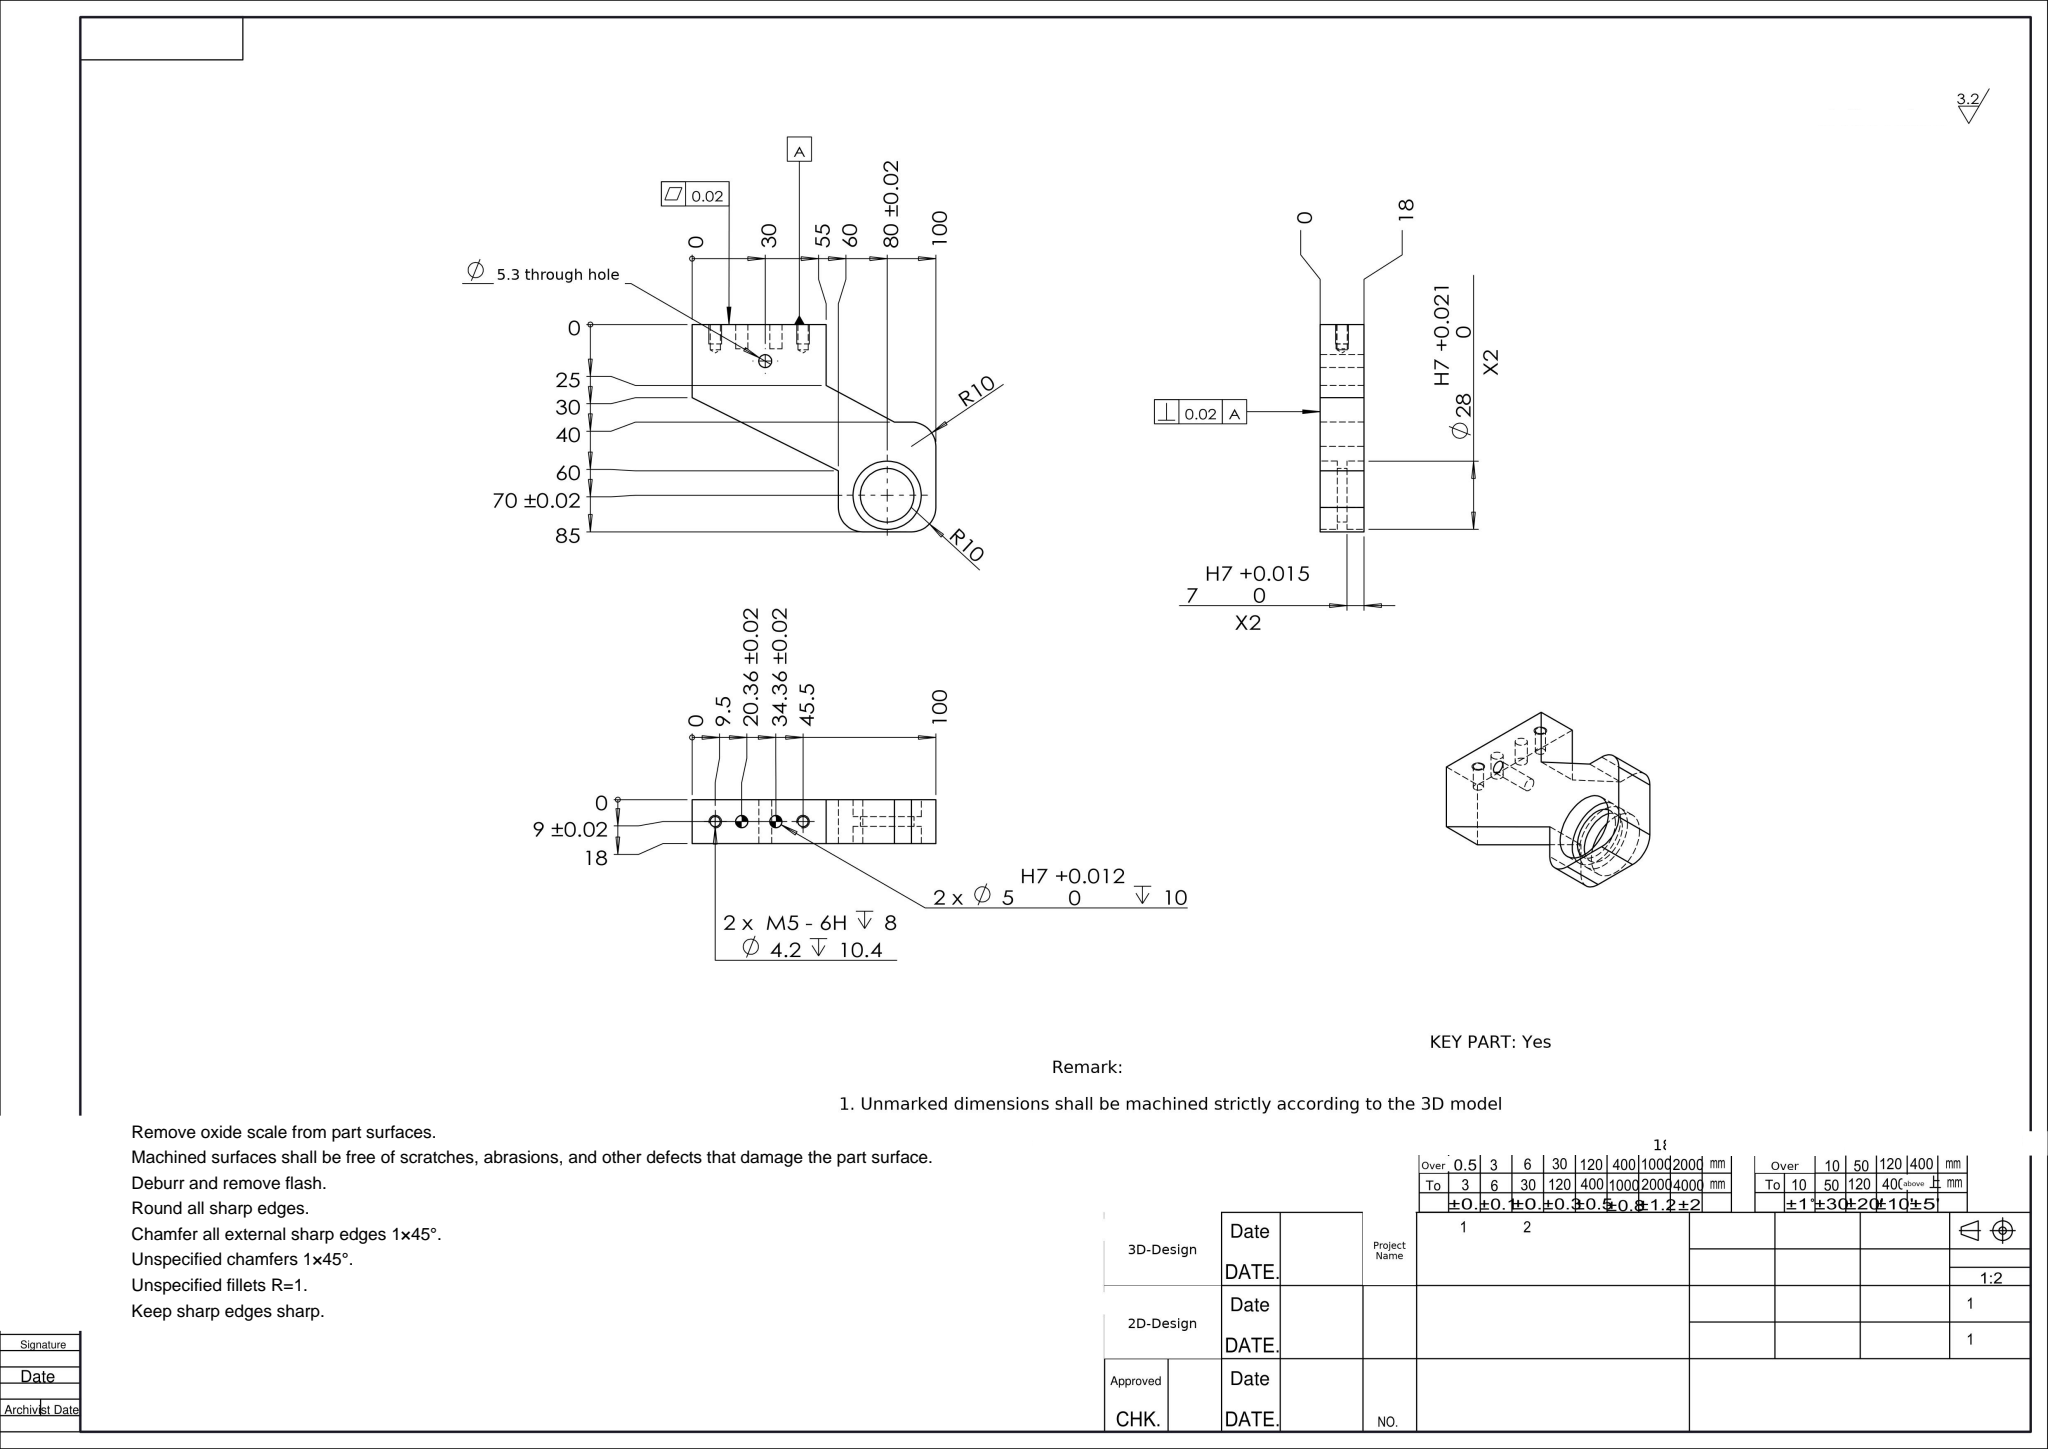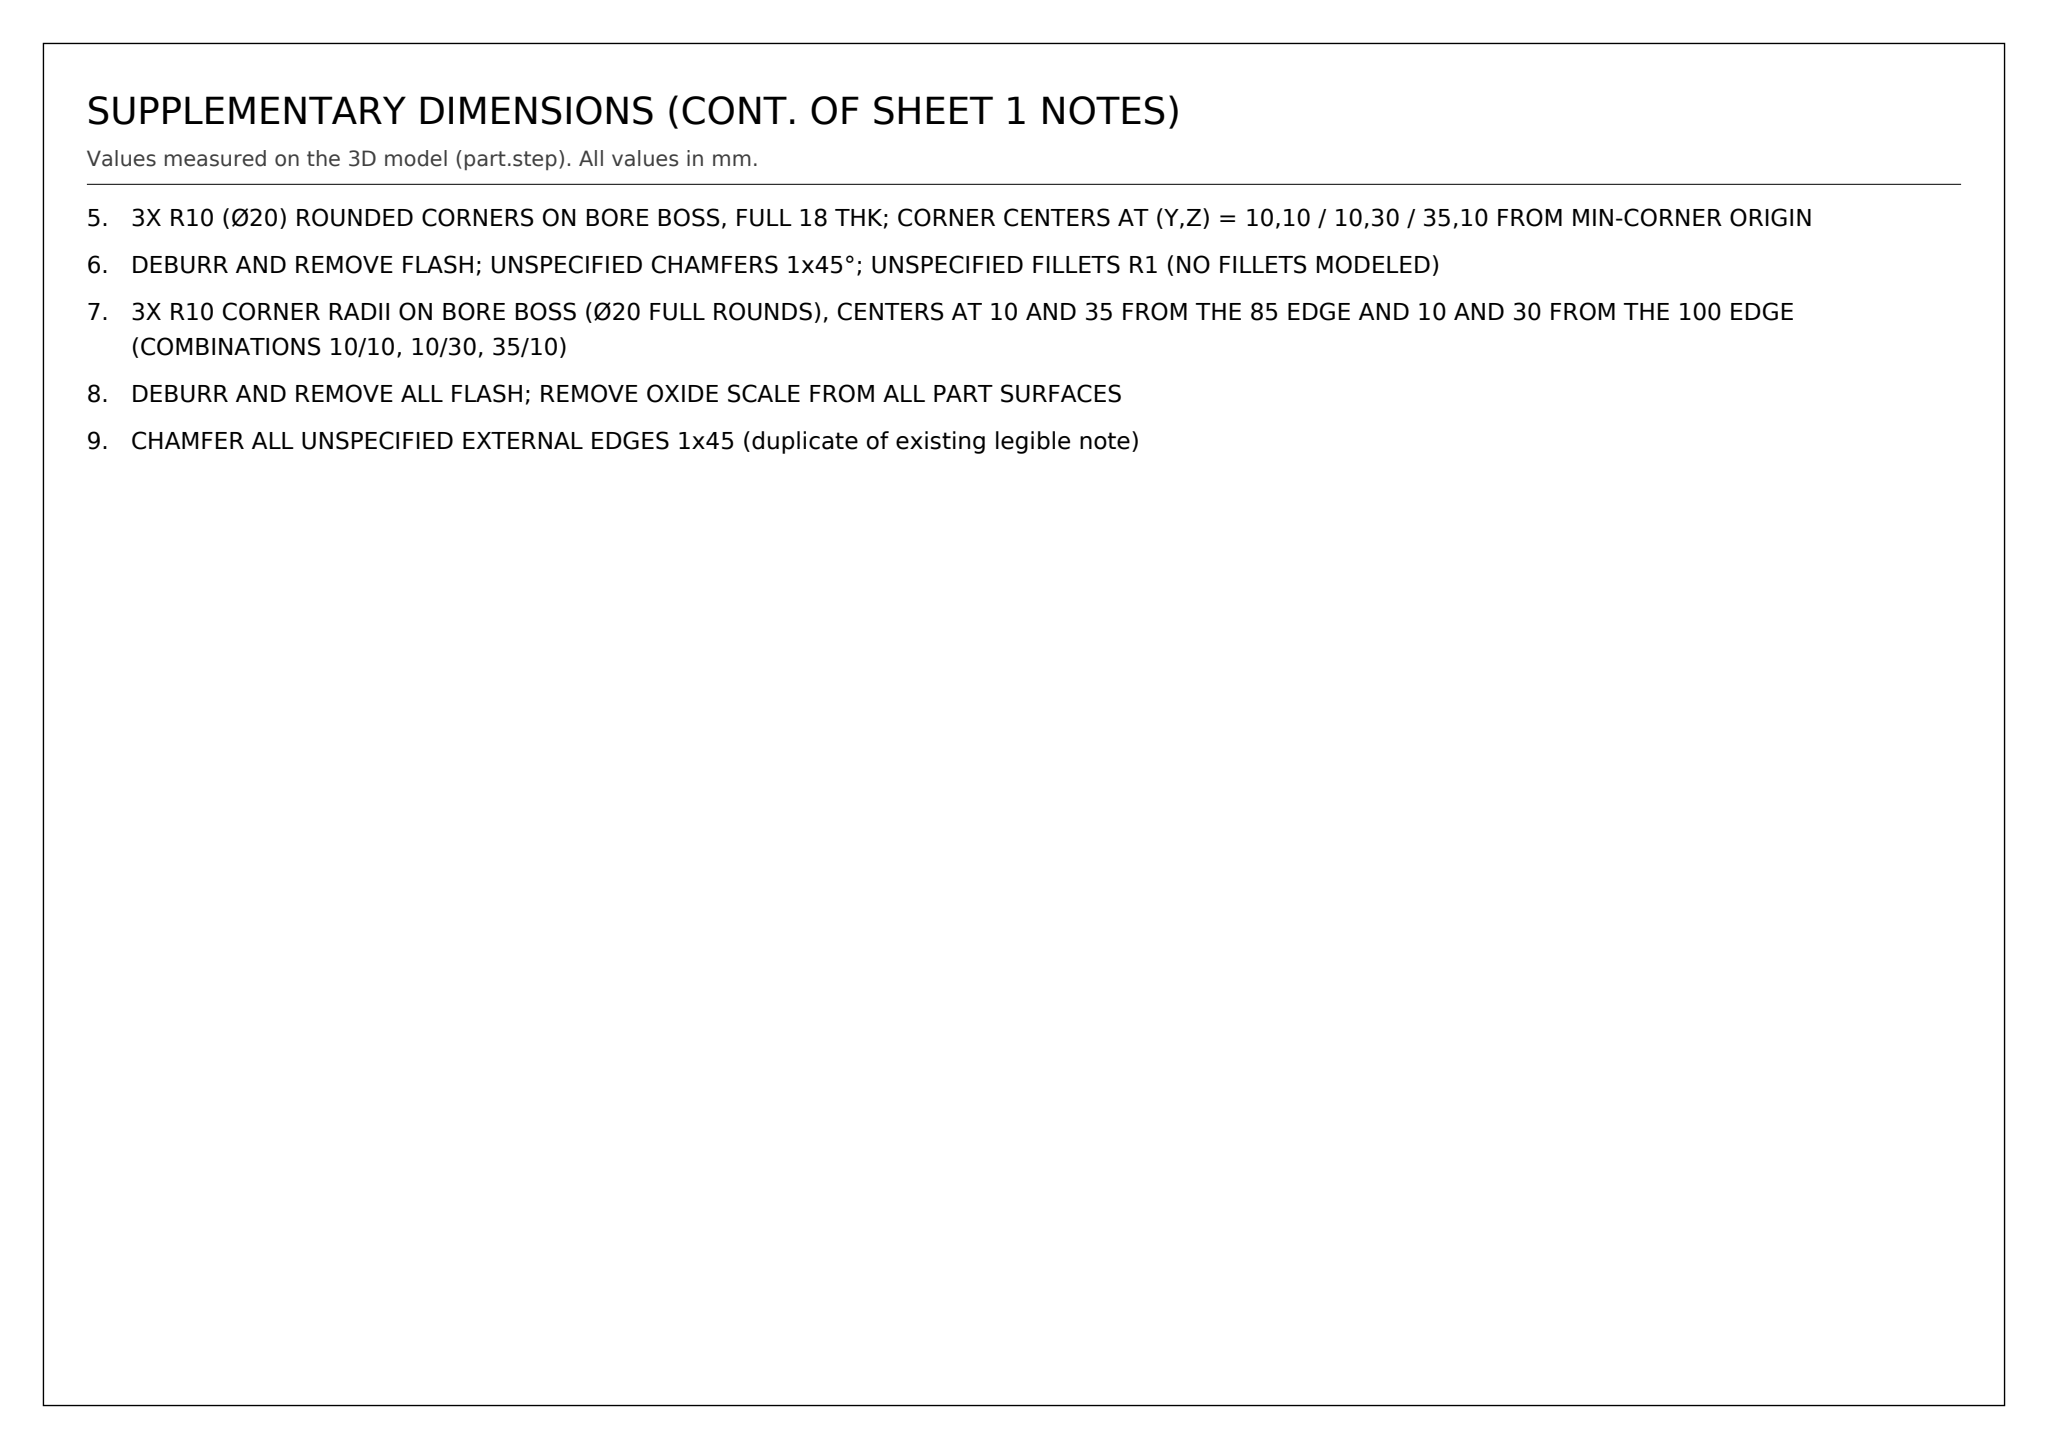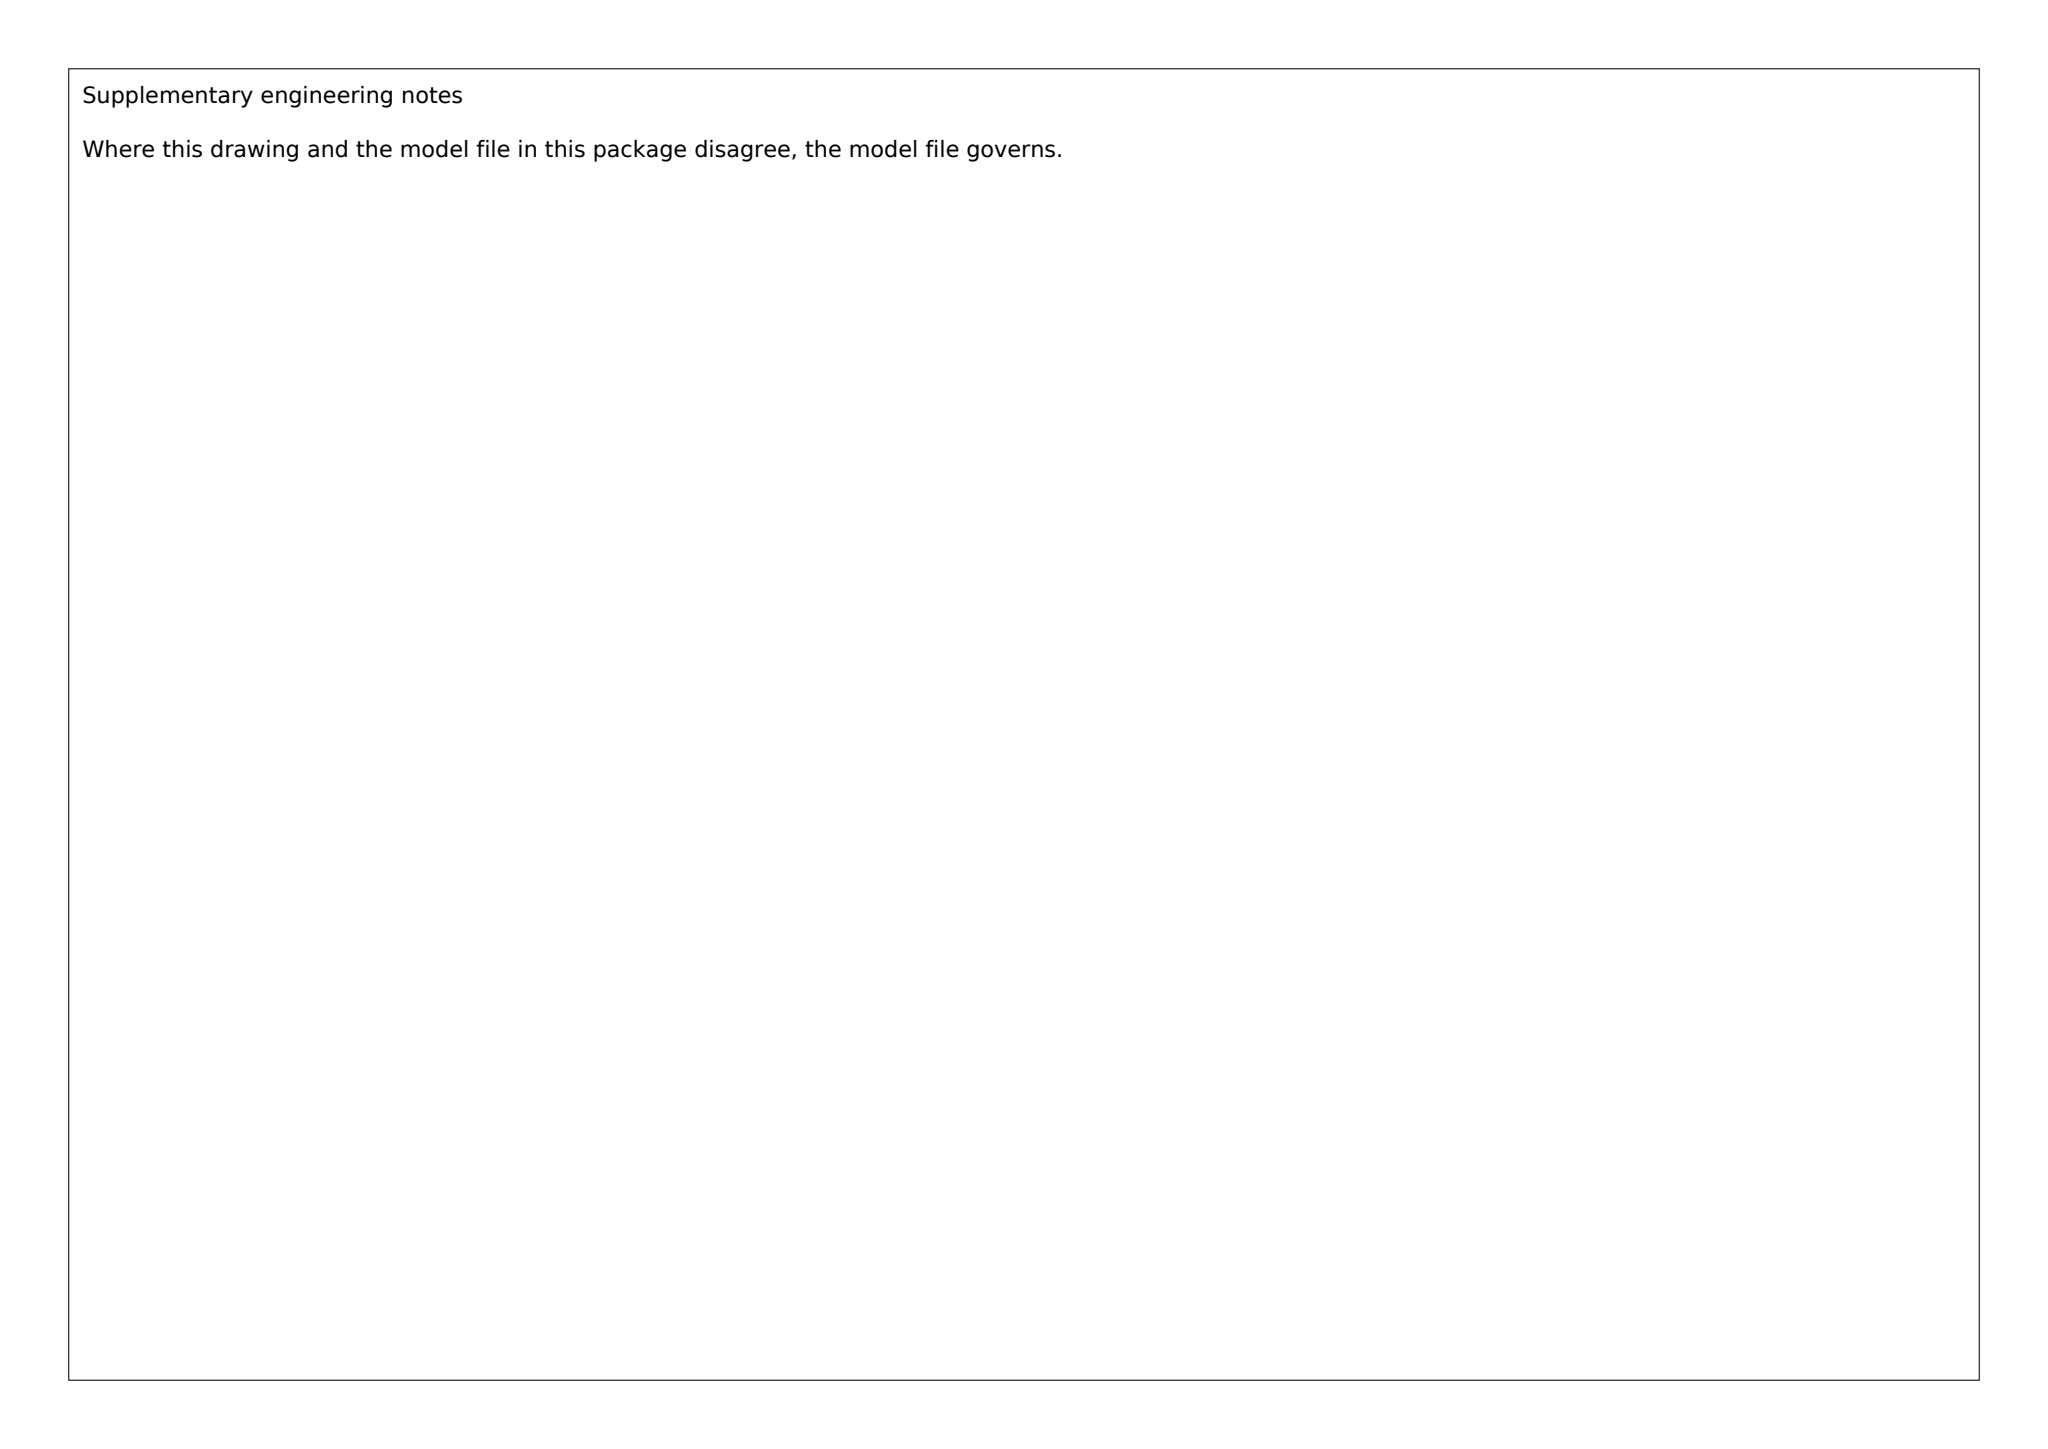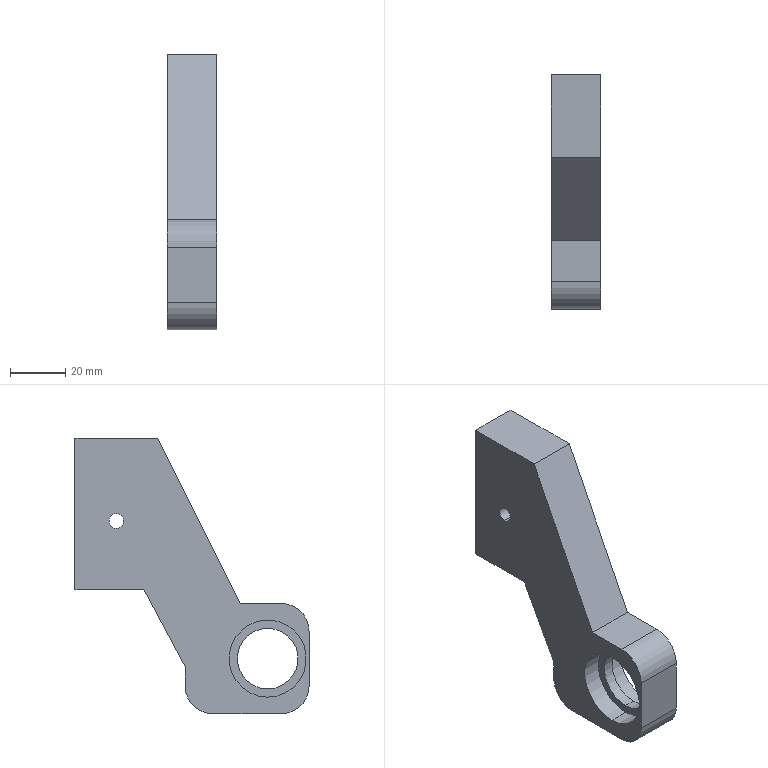Part | SolidWorks | mm | 1 solid | 38 faces | box 18 x 85 x 100 mm | volume 68790 mm3 | cylinder 19 | plane 15 | cone 4 | commonest cylinder face diameters 5 x4 4.2 x4 28 x4 20 x3 5.3 x2 22 x2
Drawing notes:
OVERALL 18 THK x 85 x 100 | from the solid: bbox_xyz 18 x 85 x 100
UPPER BOSS 18 THK FULL, NO STEP; 25/30/40/60 ARE PROFILE DIMS ONLY | from the solid: only outer x-planes 0 and 18 over boss; x=7 and 11 are Ø28 bore bottoms; bbox x=18
Ø28 H7 DP 7 EA FACE, Ø22 x 4 WIDE RELIEF BETWEEN, THRU | from the solid: dia 28 len 7 both faces + dia 22 len 4 same axis (y=15,z=20); 7+4+7=18 = thk; x-planes 0/7/11/18
Ø5.3 THRU, 30 FROM LEFT EDGE, 15 FROM TOP EDGE (FRONT VW) | from the solid: cyl dia 5.3 axis x at (y=70,z=70), len 18 = full thk; 100-70=30, 85-70=15
3X R10 (Ø20) ROUNDED CORNERS ON BORE BOSS, FULL 18 THK; CORNER CENTERS AT (Y,Z) = 10,10 / 10,30 / 35,10 FROM MIN-CORNER ORIGIN | from the solid: cylinders dia 20, axis x, length 18, at pos [y10,z10], [y10,z30], [y35,z10] (3 occurrences)
DEBURR AND REMOVE FLASH; UNSPECIFIED CHAMFERS 1x45°; UNSPECIFIED FILLETS R1 (NO FILLETS MODELED) | from the solid: fillet_radii: [] (empty)
3X R10 CORNER RADII ON BORE BOSS (Ø20 FULL ROUNDS), CENTERS AT 10 AND 35 FROM THE 85 EDGE AND 10 AND 30 FROM THE 100 EDGE (COMBINATIONS 10/10, 10/30, 35/10) | from the solid: cylinders dia 20.0 axis x at (y,z)=(10,10), (10,30), (35,10), length 18 (3 off)
DEBURR AND REMOVE ALL FLASH; REMOVE OXIDE SCALE FROM ALL PART SURFACES | from the solid: general finishing note restored after redaction of overlapping text; no STEP dimension involved
CHAMFER ALL UNSPECIFIED EXTERNAL EDGES 1x45 (duplicate of existing legible note) | from the solid: no STEP chamfer feature; text restored from redacted overlapping line only
build123d program:
from build123d import *

# Parameters (mm, degrees)
SKETCH1_W                     = 40
SKETCH1_H                     = 70
BOSS_EXTRUDE1_DEPTH           = 9
SKETCH3_W                     = 18
SKETCH3_H                     = 40
BOSS_EXTRUDE2_DEPTH           = 15
SKETCH5_R                     = 14
CUT_EXTRUDE3_DEPTH            = 7
SKETCH6_R                     = 11
CUT_EXTRUDE4_DEPTH            = 11
BOSS_EXTRUDE3_DEPTH           = 18
CUT_EXTRUDE5_DEPTH            = 18
M5_CLEARANCE_HOLE1_D          = 5.3
M5_TAPPED_HOLE1_D             = 4.2
M5_TAPPED_HOLE1_DEPTH         = 10.4
M5_TAPPED_HOLE1_TIP           = 1.262
SIZE_MM_DOWEL_PIN_HOLE1_D     = 5
SIZE_MM_DOWEL_PIN_HOLE1_DEPTH = 10
FILLET1_R                     = 10


with BuildPart() as part:
    # Sketch1 → Boss-Extrude1 (new, symmetric)
    with BuildSketch(Plane(origin=(0, 0, 0), x_dir=(0, 0, -1), z_dir=(1, 0, 0))):
        Rectangle(SKETCH1_W, SKETCH1_H)
    extrude(amount=BOSS_EXTRUDE1_DEPTH, both=True)

    # Sketch3 → Boss-Extrude2 (add)
    with BuildSketch(Plane(origin=(0, 35, 0), x_dir=(1, 0, 0), z_dir=(0, 1, 0))):
        Rectangle(SKETCH3_W, SKETCH3_H)
    extrude(amount=BOSS_EXTRUDE2_DEPTH)

    # Sketch5 → Cut-Extrude3 (cut)
    with BuildSketch(Plane(origin=(9, 0, 0), x_dir=(0, 0, -1), z_dir=(1, 0, 0))):
        with Locations((0, -20)):
            Circle(SKETCH5_R)
    cut_extrude3 = extrude(amount=-CUT_EXTRUDE3_DEPTH, mode=Mode.SUBTRACT)

    # Sketch6 → Cut-Extrude4 (cut)
    with BuildSketch(Plane(origin=(2, 0, 0), x_dir=(0, 0, -1), z_dir=(1, 0, 0))):
        with Locations((0, -20)):
            Circle(SKETCH6_R)
    extrude(amount=-CUT_EXTRUDE4_DEPTH, mode=Mode.SUBTRACT)

    # Mirror1: Cut-Extrude3 across plane
    add(cut_extrude3.mirror(Plane(origin=(0, 0, 0), x_dir=(0, 0, 1), z_dir=(1, 0, 0))), mode=Mode.SUBTRACT)

    # Sketch7 → Boss-Extrude3 (add)
    with BuildSketch(Plane.ZY.offset(9)):
        Polygon((20, 50), (80, 50), (80, 20), (20, -10), align=None)
    extrude(amount=-BOSS_EXTRUDE3_DEPTH)

    # Sketch8 → Cut-Extrude5 (cut)
    with BuildSketch(Plane.ZY.offset(9)):
        Polygon((-20, 50), (-20, 10), (-3, 10), (25, 25), (25, 50), align=None)
    extrude(amount=-CUT_EXTRUDE5_DEPTH, mode=Mode.SUBTRACT)

    # M5 Clearance Hole1 (through all)
    with Locations(Plane(origin=(9, 0, 0), x_dir=(0, 0, -1), z_dir=(1, 0, 0))):
        with Locations((-50, 35)):
            Hole(M5_CLEARANCE_HOLE1_D / 2)

    # M5 Tapped Hole1
    with Locations(Plane(origin=(0, 50, 0), x_dir=(1, 0, 0), z_dir=(0, 1, 0))):
        with Locations((0, -34.5), (0, -70.5)):
            Hole(M5_TAPPED_HOLE1_D / 2, depth=M5_TAPPED_HOLE1_DEPTH)
            with Locations((0, 0, -(M5_TAPPED_HOLE1_DEPTH + M5_TAPPED_HOLE1_TIP / 2))):  # 118° drill point
                Cone(0, M5_TAPPED_HOLE1_D / 2, M5_TAPPED_HOLE1_TIP, mode=Mode.SUBTRACT)

    # Size mm Dowel Pin Hole1
    with Locations(Plane(origin=(0, 50, 0), x_dir=(1, 0, 0), z_dir=(0, 1, 0))):
        with Locations((0, -45.64), (0, -59.64)):
            Hole(SIZE_MM_DOWEL_PIN_HOLE1_D / 2, depth=SIZE_MM_DOWEL_PIN_HOLE1_DEPTH)

    # Fillet1
    fillet1_edges = [part.edges().sort_by_distance(p)[0] for p in [
        (0, 10, -20),
        (0, -35, -20),
        (0, -35, 20),
    ]]
    fillet(fillet1_edges, radius=FILLET1_R)


solid = part.part